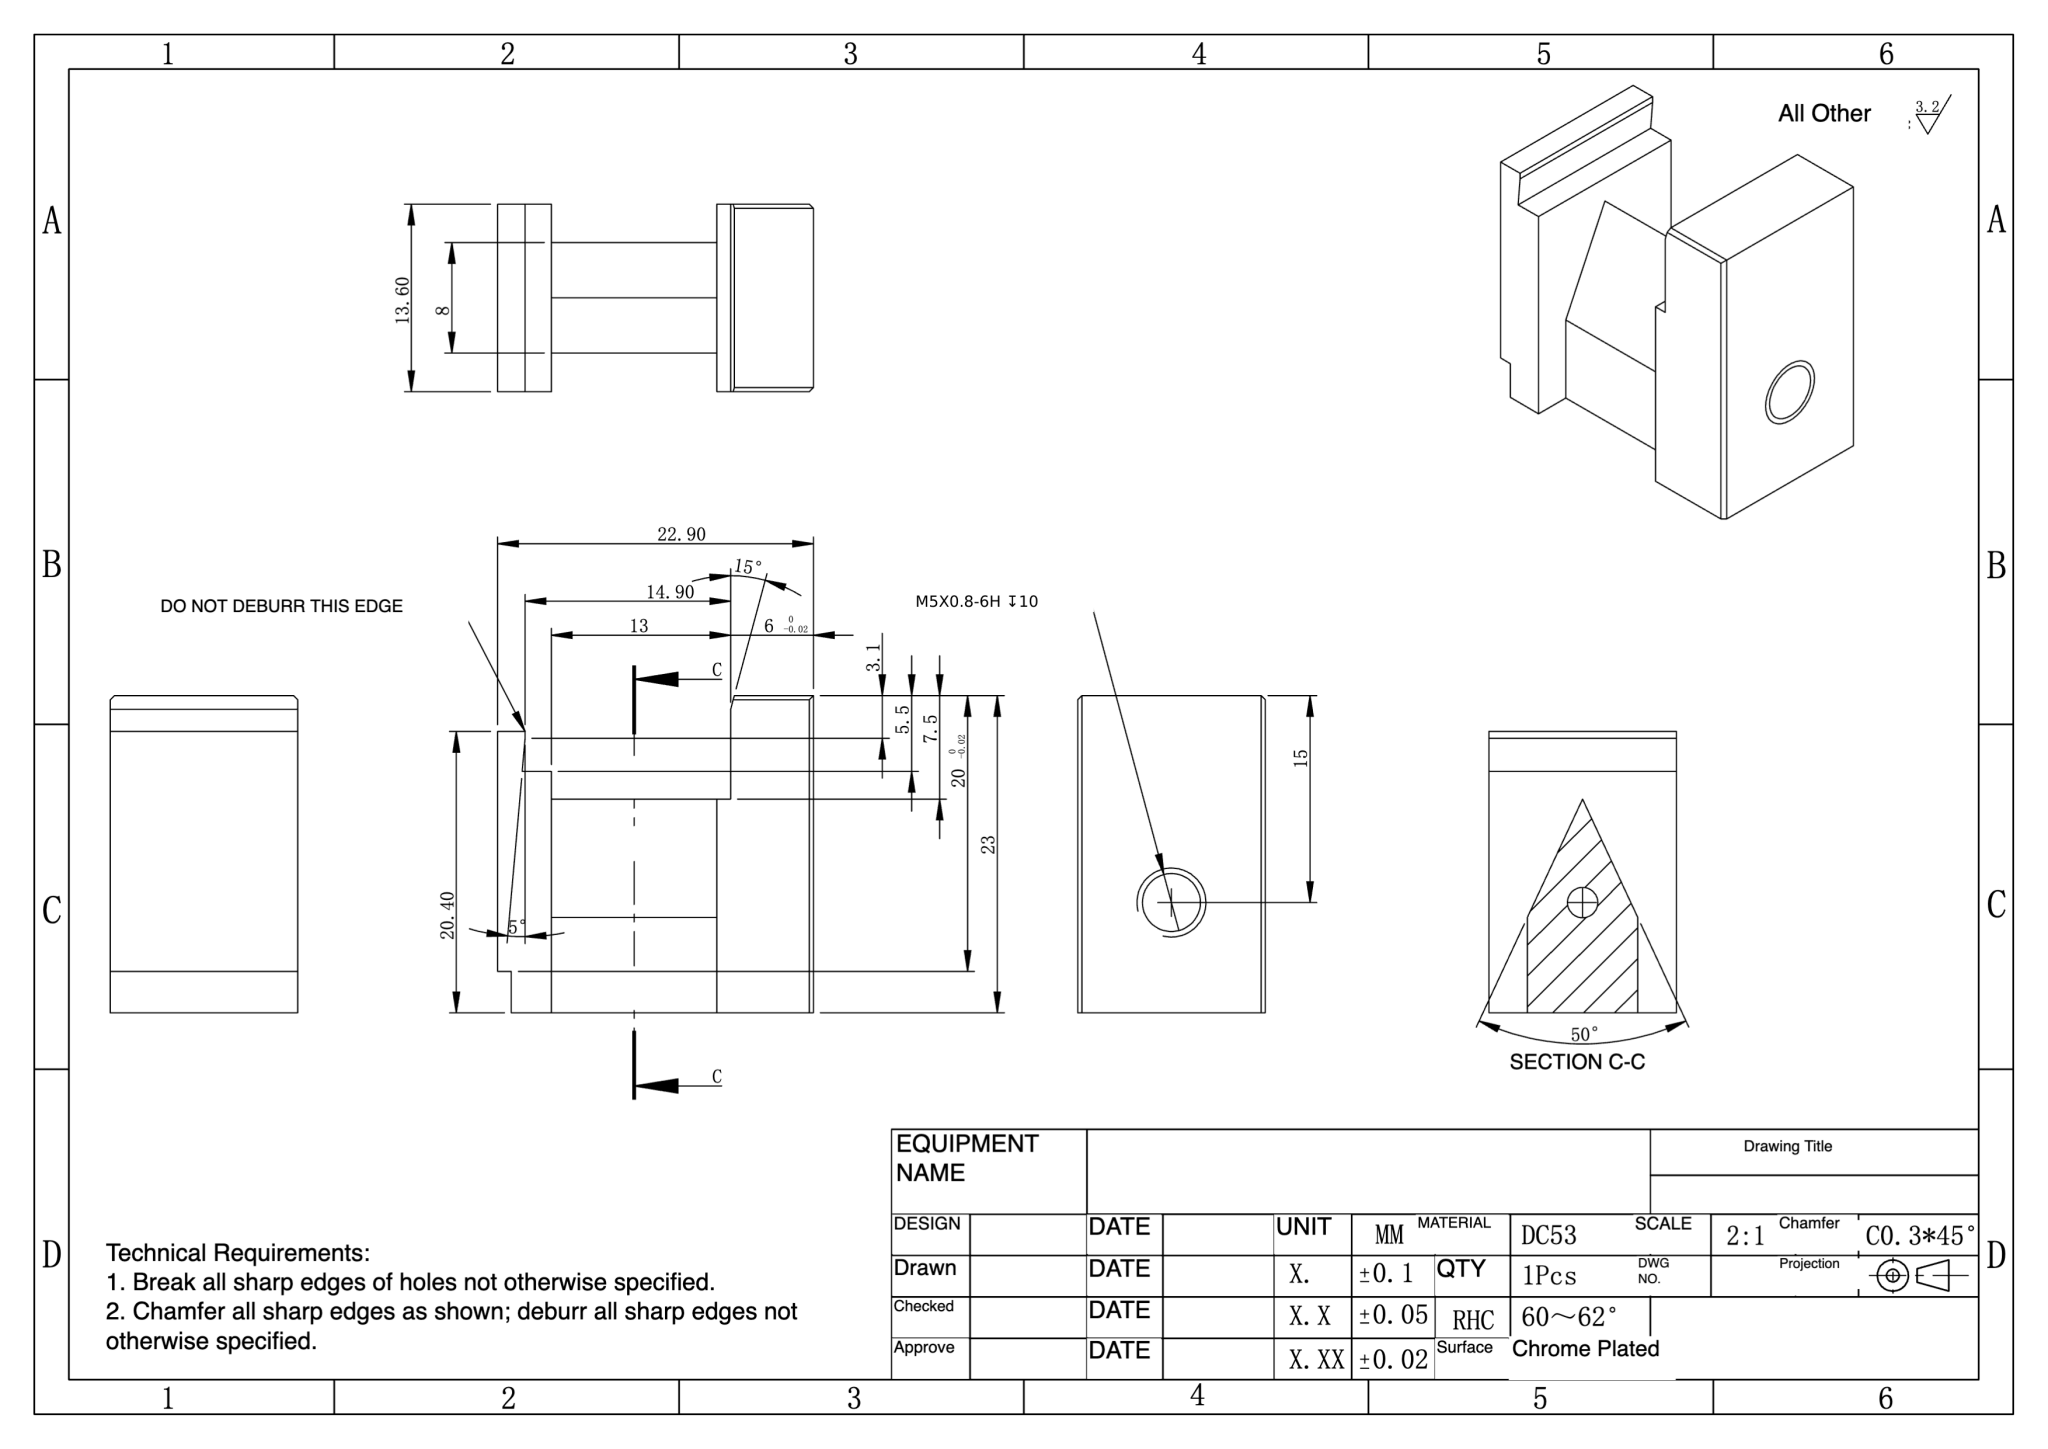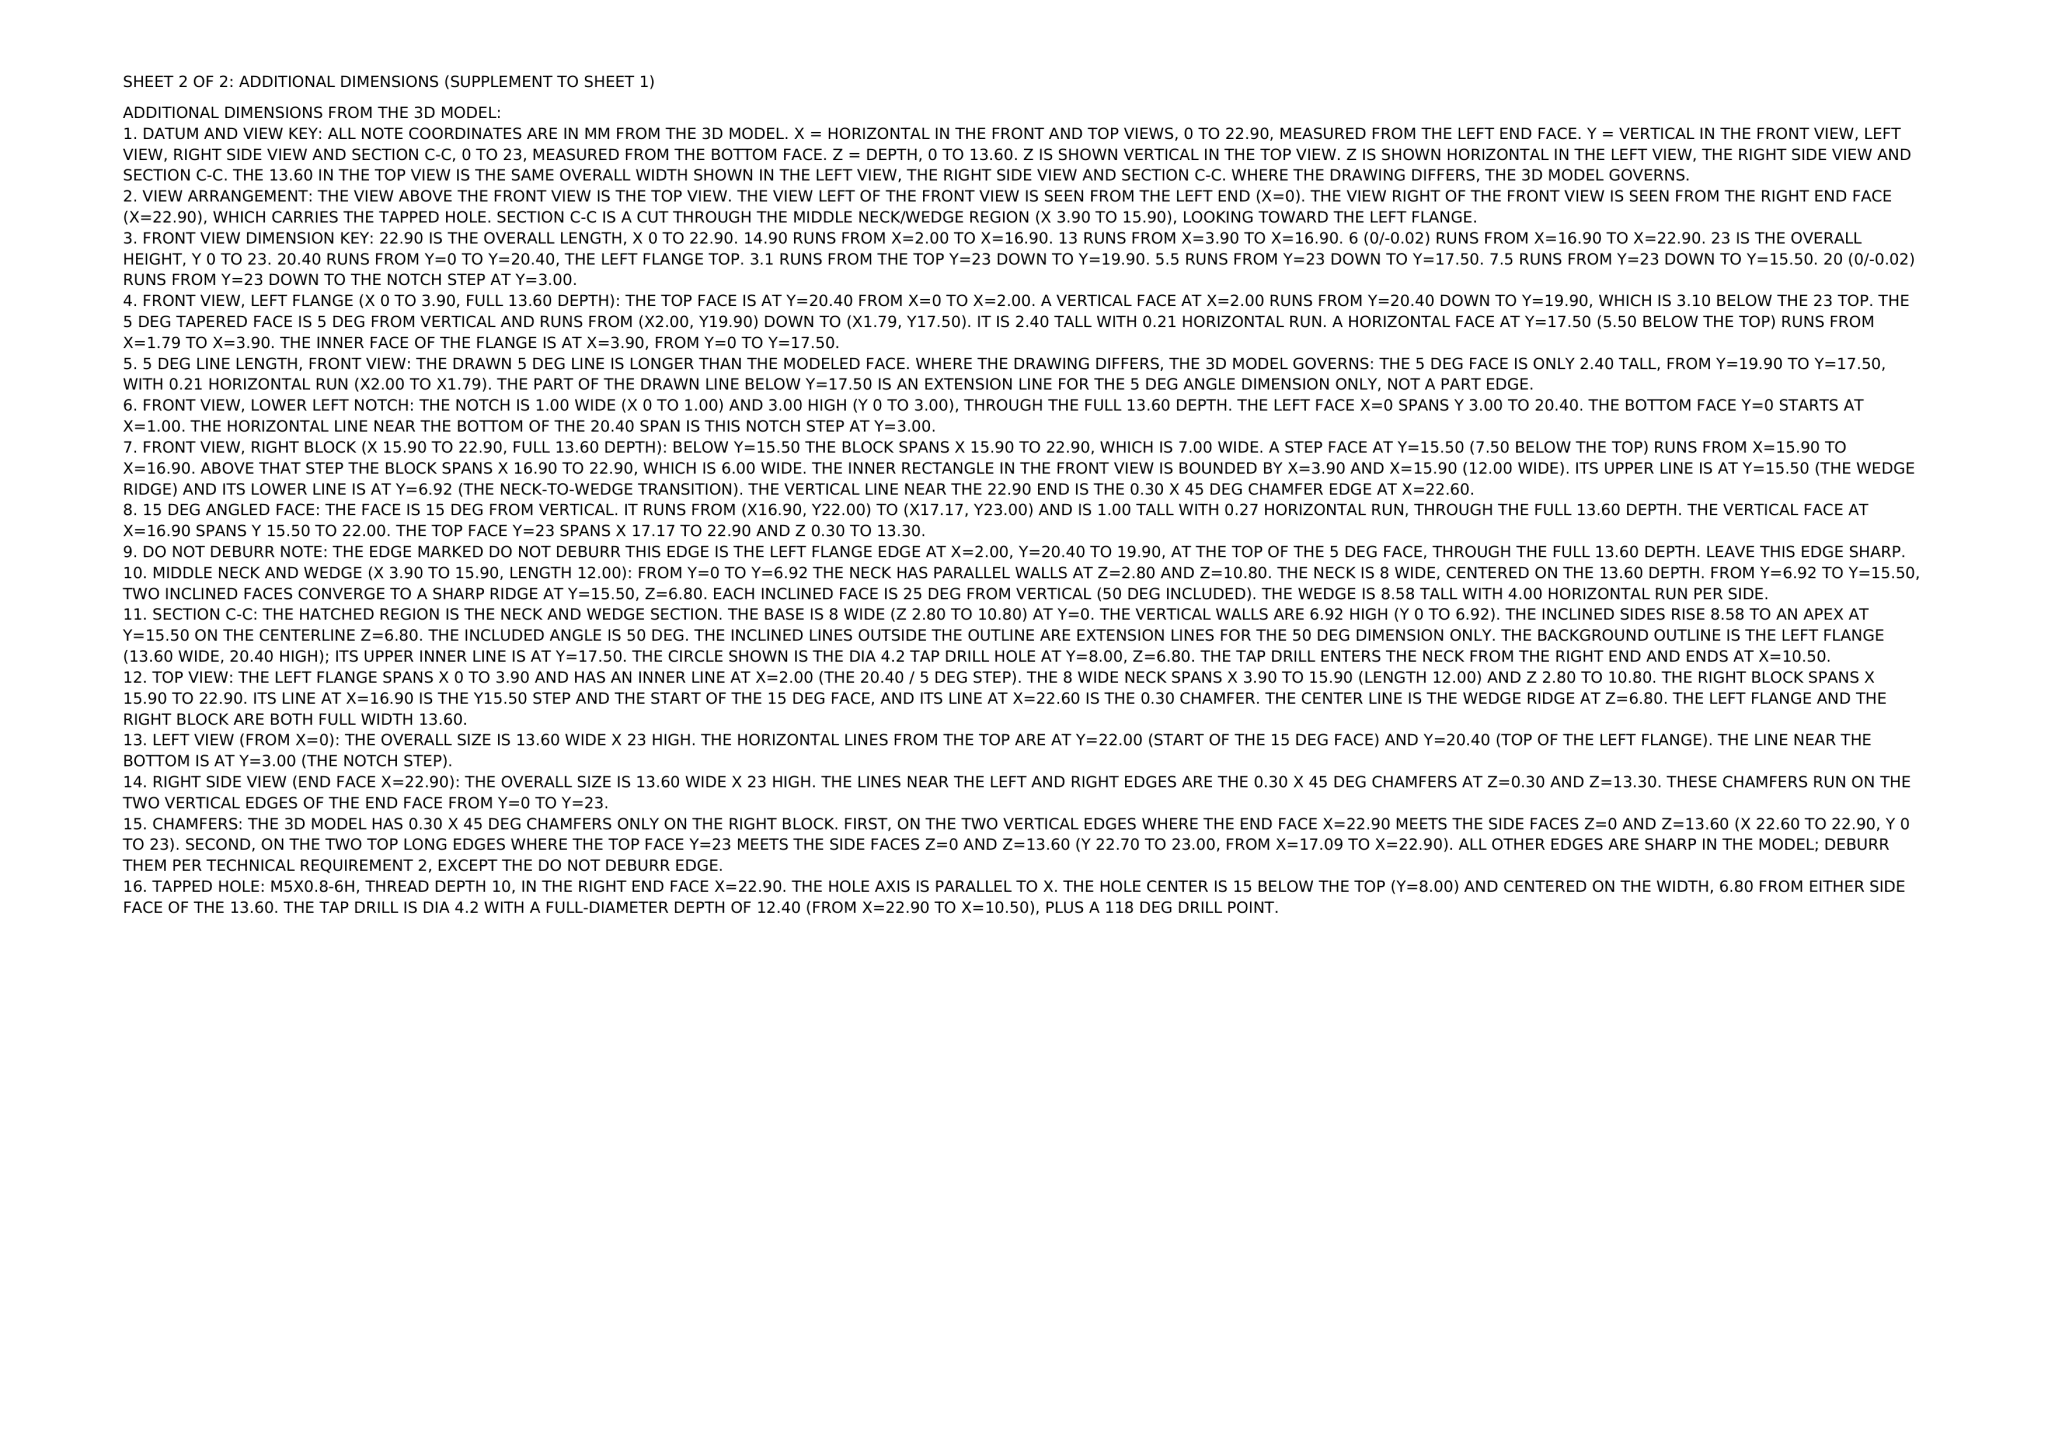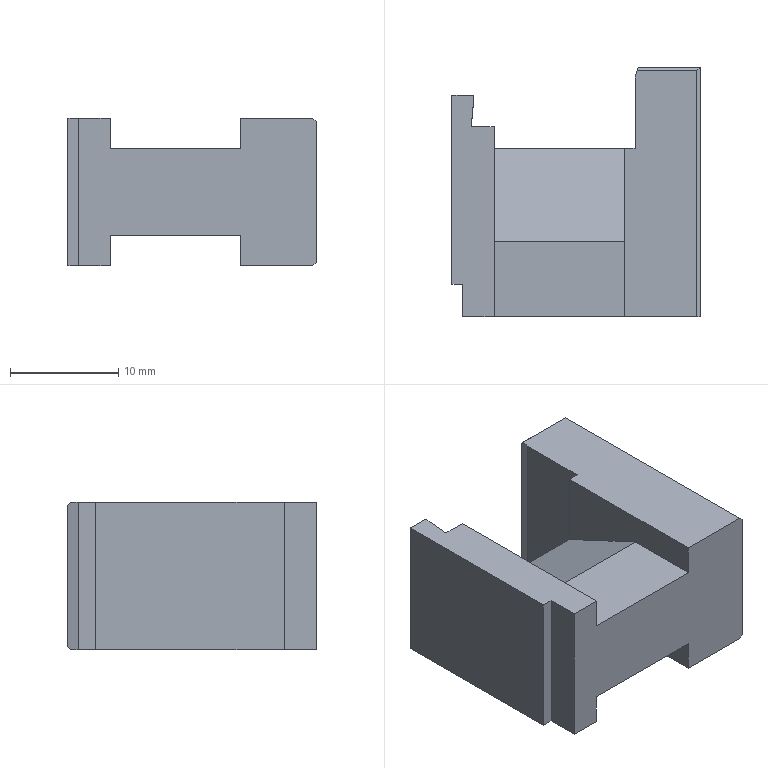Part | NX | mm | Slotted Slide Block | 1 solid | 32 faces | box 22.9 x 23 x 13.6 mm | volume 3945 mm3 | plane 28 | cylinder 2 | cone 2 | commonest cylinder face diameters 4.2 x2